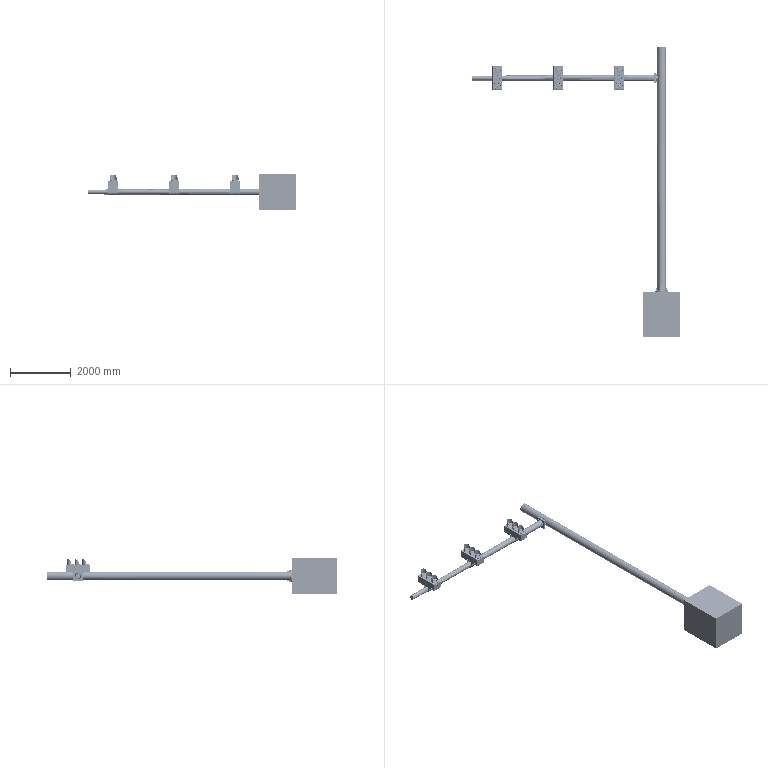Assembly | SolidWorks | mm | 155 component files | 155 solids | 5469 faces | box 6816.5 x 9530 x 1200 mm | volume 2287948976 mm3 | cylinder 2731 | plane 1552 | cone 624 | spline 470 | torus 92 | commonest cylinder face diameters 5 x1476 8 x192 9 x180 10 x168 6 x108 2 x72 15 x72 7 x72
Bill of materials:
Accessory1 | 3 |  | U-shaped thin-wall channel or saddle: a semicircular trough with straight vertical side walls ending in two flat outward flanges, each with two small through-holes.
Base | 1 |  | Plain rectangular block with a row of small cylindrical pins sticking out of one face.
Cantilever | 1 |  | Long, slender round tube with a square end plate at one end. The plate has a central circular opening and four corner holes.
Cap | 1 |  | Short cylindrical cup or cap: a thin-walled ring closed at one end by a flat disc.
Column | 1 |  | Long round tube with a circular bolt-hole flange at one end and a small rectangular tab or bracket plate attached near the other end.
GB_T5786-2000[HexHeadBoltFineThreadFullThreadM16_1.5_70] | 4 |  | Hex-head bolt-like part: a hexagonal head with a long, plain cylindrical shank. The shank's free end is chamfered.
GB_T6170-2015[Type1HexNutM16] | 4 |  | Hex nut-like part: a hexagonal prism with a central through-bore and chamfered corners on both faces.
GB_T6170-2015[Type1HexNutM24] | 8 |  | Hex nut-like part: a hexagonal prism with a central through-bore and double-sided corner chamfers. It looks almost the same as unnamed part.
HexFlangeBoltM10x25 | 12 |  | Hex flange-head bolt or screw: a hexagonal head with an integral round flange washer and a plain cylindrical shank.
HexNutM10 | 12 |  | Hexagonal nut with a plain central through-bore and chamfered corners on both faces.
CoverPlate | 3 |  | Shallow rectangular tray or pan: a flat base with a low wall around all four sides and several through-holes in the base.
GreenLight | 3 |  | Round cap or plug: a slightly domed disc with a thin rim, over a tapered underside that steps down to a smaller cylindrical spigot.
LampHolderMountingPlate | 36 |  | Bent sheet bracket or gusset: a roughly trapezoidal or pentagonal flat plate with one large hole, plus a narrow flange bent up along one curved edge.
Lampshade | 9 |  | Thin curved sheet shroud: a partial cylinder (open arc of about 180-200 degrees) with a curved, sloped top edge and small holes near the bottom edge.
LightBox | 3 |  | Rectangular box-shaped housing. The top face has three large round openings, each surrounded by a pattern of small holes. One end face has a round boss with a hole. The edges are slightly rounded, and there is a recessed lip or panel at the base.
LightMountingPlate | 9 |  | Flat annular ring (washer/flange-like) with four evenly spaced axial through holes, a small radial pin protruding from the outer rim, and a small radial hole in the outer cylindrical face.
OuterFrame | 3 |  | Thin, flat rectangular open frame made of four narrow rails of the same width around a large rectangular opening; the outline is roughly 2.7 times as long as it is wide.
RedLight | 3 |  | Round cap or knob-like solid: a slightly domed top face, a thin cylindrical rim, an underside that curves and tapers inward, and a smaller cylindrical boss at the bottom.
Screw1 | 36 |  | Stepped, rotationally symmetric part: a hollow cylindrical tip with an open bore at the top, a middle step, a larger cylindrical collar, a short plain neck, and a threaded shank modelled with visible thread grooves.
YellowLight | 3 |  | Round cap or knob-like solid: a slightly domed top face, a thin cylindrical rim, an underside that curves and tapers inward, and a cylindrical boss at the bottom.
Mates:
1. concentric | Column-1 face at (-142.894, -198, 82.5) dir (0, 1, 0) r 12 | Base-1 face at (-142.894, 50, 82.5) dir (0, -1, 0) r 12
2. concentric | Column-1 face at (-42.705, -198, 159.378) dir (0, 1, 0) r 12 | Base-1 face at (-42.705, 50, 159.378) dir (0, -1, 0) r 12
3. coincident | Column-1 face at (0, 0, 0) dir (0, -1, 0) | Base-1 face at (0, 0, 0) dir (0, 1, 0)
4. coincident | Column-1 face at (0, 20, 0) dir (0, 1, 0) | GB_T6170-2015[Type1HexNutM24]-1 face at (-142.894, 20, 61.715) dir (0, -1, 0)
5. concentric | Cantilever-1 face at (-6216.5, 7000, 0) dir (-1, 0, 0) r 4.667 | Column-1 face at (206.501, 7000, 0) dir (-1, 0, 0) r 80
6. concentric | Column-1 face at (-186.5, 7106.066, 106.066) dir (-1, 0, 0) r 8 | Cantilever-1 face at (-216.5, 7106.066, 106.066) dir (-1, 0, 0) r 8
7. coincident | Column-1 face at (-216.5, 0, 0) dir (-1, 0, 0) | Cantilever-1 face at (-216.5, 7000, 0) dir (1, 0, 0)
8. concentric | Column-1 face at (-186.5, 7106.066, 106.066) dir (-1, 0, 0) r 8 | GB_T5786-2000[HexHeadBoltFineThreadFullThreadM16_1.5_70]-1 face at (-176.5, 7106.066, 106.066) dir (1, 0, 0) r 8
9. coincident | Column-1 face at (-186.5, 0, 0) dir (1, 0, 0) | GB_T5786-2000[HexHeadBoltFineThreadFullThreadM16_1.5_70]-1 face at (-186.5, 7128.247, 115.23) dir (-1, 0, 0)
10. coincident | Cantilever-1 face at (-236.5, 2747.057, -6675.305) dir (-1, 0, 0) | GB_T6170-2015[Type1HexNutM16]-1 face at (-236.5, 7119.922, 106.066) dir (1, 0, 0)
11. concentric | Column-1 face at (0, 8020, 0) dir (0, -1, 0) r 136.5 | Cap-1 face at (0, 7920, 0) dir (0, 1, 0) r 146.5
12. coincident | Column-1 face at (0, 8020, 0) dir (0, 1, 0) | Cap-1 face at (0, 8020, 0) dir (0, -1, 0)
13. parallel | Cap-1 face at (0, 8030, 0) dir (0, 1, 0) | Light-1/LightBox-1 face at (-5543.393, 7384.024, 358.679) dir (0, 1, 0)
14. parallel | Base-1 face at (-600, -1500, -600) dir (0, 0, -1) | Light-1/CoverPlate-1 face at (-5543.955, 7380.024, 119.592) dir (0, 0, -1)
15. concentric | Light-1/CoverPlate-1 face at (-5301.127, 7146.665, 489.592) dir (0, 0, -1) r 5 | Accessory1-1 face at (-5301.127, 7146.665, 479.592) dir (0, 0, -1) r 5
16. coincident | Light-1/CoverPlate-1 face at (-5543.955, 7380.024, 119.592) dir (0, 0, -1) | Accessory1-1 face at (-5123.37, 7112.081, 119.592) dir (0, 0, 1)
17. coincident | Accessory1-1 face at (-5162.522, 7112.081, 109.592) dir (0, 0, -1) | HexFlangeBoltM10x25-1 plane at (-5489.995, 7146.665, 109.592) dir (0, 0, 1)
18. concentric | Accessory1-1 face at (-5489.995, 7146.665, 479.592) dir (0, 0, -1) r 5 | HexFlangeBoltM10x25-1 axis at (-5489.995, 7146.665, 109.592) dir (0, 0, 1)
19. coincident | Accessory1-1 face at (-5162.522, 7112.081, 109.592) dir (0, 0, -1) | HexFlangeBoltM10x25-2 plane at (-5301.127, 7146.665, 109.592) dir (0, 0, 1)
20. concentric | Accessory1-1 face at (-5301.127, 7146.665, 479.592) dir (0, 0, -1) r 5 | HexFlangeBoltM10x25-2 axis at (-5301.127, 7146.665, 109.592) dir (0, 0, 1)
21. coincident | Accessory1-1 face at (-5162.522, 7112.081, 109.592) dir (0, 0, -1) | HexFlangeBoltM10x25-3 plane at (-5301.127, 6853.335, 109.592) dir (0, 0, 1)
22. concentric | Accessory1-1 face at (-5301.127, 6853.335, 479.592) dir (0, 0, -1) r 5 | HexFlangeBoltM10x25-3 axis at (-5301.127, 6853.335, 109.592) dir (0, 0, 1)
23. coincident | Accessory1-1 face at (-5162.522, 7112.081, 109.592) dir (0, 0, -1) | HexFlangeBoltM10x25-4 plane at (-5489.995, 6853.335, 109.592) dir (0, 0, 1)
24. concentric | Accessory1-1 face at (-5489.995, 6853.335, 479.592) dir (0, 0, -1) r 5 | HexFlangeBoltM10x25-4 axis at (-5489.995, 6853.335, 109.592) dir (0, 0, 1)
25. coincident | Accessory1-2 face at (-3162.522, 7112.081, 109.592) dir (0, 0, -1) | HexFlangeBoltM10x25-5 plane at (-3489.995, 7146.665, 109.592) dir (0, 0, 1)
26. concentric | Accessory1-2 face at (-3489.995, 7146.665, 479.592) dir (0, 0, -1) r 5 | HexFlangeBoltM10x25-5 axis at (-3489.995, 7146.665, 109.592) dir (0, 0, 1)
27. coincident | Accessory1-2 face at (-3162.522, 7112.081, 109.592) dir (0, 0, -1) | HexFlangeBoltM10x25-6 plane at (-3301.127, 7146.665, 109.592) dir (0, 0, 1)
28. concentric | Accessory1-2 face at (-3301.127, 7146.665, 479.592) dir (0, 0, -1) r 5 | HexFlangeBoltM10x25-6 axis at (-3301.127, 7146.665, 109.592) dir (0, 0, 1)
29. coincident | Accessory1-2 face at (-3162.522, 7112.081, 109.592) dir (0, 0, -1) | HexFlangeBoltM10x25-7 plane at (-3301.127, 6853.335, 109.592) dir (0, 0, 1)
30. concentric | Accessory1-2 face at (-3301.127, 6853.335, 479.592) dir (0, 0, -1) r 5 | HexFlangeBoltM10x25-7 axis at (-3301.127, 6853.335, 109.592) dir (0, 0, 1)
31. coincident | Accessory1-2 face at (-3162.522, 7112.081, 109.592) dir (0, 0, -1) | HexFlangeBoltM10x25-8 plane at (-3489.995, 6853.335, 109.592) dir (0, 0, 1)
32. concentric | Accessory1-2 face at (-3489.995, 6853.335, 479.592) dir (0, 0, -1) r 5 | HexFlangeBoltM10x25-8 axis at (-3489.995, 6853.335, 109.592) dir (0, 0, 1)
33. coincident | Accessory1-3 face at (-1162.522, 7112.081, 109.592) dir (0, 0, -1) | HexFlangeBoltM10x25-9 plane at (-1489.995, 7146.665, 109.592) dir (0, 0, 1)
34. concentric | Accessory1-3 face at (-1489.995, 7146.665, 479.592) dir (0, 0, -1) r 5 | HexFlangeBoltM10x25-9 axis at (-1489.995, 7146.665, 109.592) dir (0, 0, 1)
35. coincident | Accessory1-3 face at (-1162.522, 7112.081, 109.592) dir (0, 0, -1) | HexFlangeBoltM10x25-10 plane at (-1301.127, 7146.665, 109.592) dir (0, 0, 1)
36. concentric | Accessory1-3 face at (-1301.127, 7146.665, 479.592) dir (0, 0, -1) r 5 | HexFlangeBoltM10x25-10 axis at (-1301.127, 7146.665, 109.592) dir (0, 0, 1)
37. coincident | Accessory1-3 face at (-1162.522, 7112.081, 109.592) dir (0, 0, -1) | HexFlangeBoltM10x25-11 plane at (-1301.127, 6853.335, 109.592) dir (0, 0, 1)
38. concentric | Accessory1-3 face at (-1301.127, 6853.335, 479.592) dir (0, 0, -1) r 5 | HexFlangeBoltM10x25-11 axis at (-1301.127, 6853.335, 109.592) dir (0, 0, 1)
39. coincident | Accessory1-3 face at (-1162.522, 7112.081, 109.592) dir (0, 0, -1) | HexFlangeBoltM10x25-12 plane at (-1489.995, 6853.335, 109.592) dir (0, 0, 1)
40. concentric | Accessory1-3 face at (-1489.995, 6853.335, 479.592) dir (0, 0, -1) r 5 | HexFlangeBoltM10x25-12 axis at (-1489.995, 6853.335, 109.592) dir (0, 0, 1)
41. coincident | Light-1/CoverPlate-1 face at (-5543.955, 7380.024, 122.592) dir (0, 0, 1) | HexNutM10-10 plane at (-5301.127, 7146.665, 122.592) dir (0, 0, -1)
42. concentric | HexFlangeBoltM10x25-2 face at (-5301.127, 7146.665, 134.592) dir (0, 0, -1) r 5 | HexNutM10-10 axis at (-5301.127, 7146.665, 122.592) dir (0, 0, 1)
43. coincident | Light-1/CoverPlate-1 face at (-5543.955, 7380.024, 122.592) dir (0, 0, 1) | HexNutM10-11 plane at (-5489.995, 7146.665, 122.592) dir (0, 0, -1)
44. concentric | HexFlangeBoltM10x25-1 face at (-5489.995, 7146.665, 134.592) dir (0, 0, -1) r 5 | HexNutM10-11 axis at (-5489.995, 7146.665, 122.592) dir (0, 0, 1)
45. coincident | Light-1/CoverPlate-1 face at (-5543.955, 7380.024, 122.592) dir (0, 0, 1) | HexNutM10-12 plane at (-5489.995, 6853.335, 122.592) dir (0, 0, -1)
46. concentric | HexFlangeBoltM10x25-4 face at (-5489.995, 6853.335, 134.592) dir (0, 0, -1) r 5 | HexNutM10-12 axis at (-5489.995, 6853.335, 122.592) dir (0, 0, 1)
47. coincident | Light-1/CoverPlate-1 face at (-5543.955, 7380.024, 122.592) dir (0, 0, 1) | HexNutM10-13 plane at (-5301.127, 6853.335, 122.592) dir (0, 0, -1)
48. concentric | HexFlangeBoltM10x25-3 face at (-5301.127, 6853.335, 134.592) dir (0, 0, -1) r 5 | HexNutM10-13 axis at (-5301.127, 6853.335, 122.592) dir (0, 0, 1)
49. coincident | Light-2/CoverPlate-1 face at (-3543.955, 7380.024, 122.592) dir (0, 0, 1) | HexNutM10-14 plane at (-3489.995, 7146.665, 122.592) dir (0, 0, -1)
50. concentric | HexFlangeBoltM10x25-5 face at (-3489.995, 7146.665, 134.592) dir (0, 0, -1) r 5 | HexNutM10-14 axis at (-3489.995, 7146.665, 122.592) dir (0, 0, 1)
51. coincident | Light-2/CoverPlate-1 face at (-3543.955, 7380.024, 122.592) dir (0, 0, 1) | HexNutM10-15 plane at (-3301.127, 7146.665, 122.592) dir (0, 0, -1)
52. concentric | HexFlangeBoltM10x25-6 face at (-3301.127, 7146.665, 134.592) dir (0, 0, -1) r 5 | HexNutM10-15 axis at (-3301.127, 7146.665, 122.592) dir (0, 0, 1)
53. coincident | Light-2/CoverPlate-1 face at (-3543.955, 7380.024, 122.592) dir (0, 0, 1) | HexNutM10-16 plane at (-3301.127, 6853.335, 122.592) dir (0, 0, -1)
54. concentric | HexFlangeBoltM10x25-7 face at (-3301.127, 6853.335, 134.592) dir (0, 0, -1) r 5 | HexNutM10-16 axis at (-3301.127, 6853.335, 122.592) dir (0, 0, 1)
55. coincident | Light-2/CoverPlate-1 face at (-3543.955, 7380.024, 122.592) dir (0, 0, 1) | HexNutM10-17 plane at (-3489.995, 6853.335, 122.592) dir (0, 0, -1)
56. concentric | HexFlangeBoltM10x25-8 face at (-3489.995, 6853.335, 134.592) dir (0, 0, -1) r 5 | HexNutM10-17 axis at (-3489.995, 6853.335, 122.592) dir (0, 0, 1)
57. coincident | Light-3/CoverPlate-1 face at (-1543.955, 7380.024, 122.592) dir (0, 0, 1) | HexNutM10-18 plane at (-1489.995, 7146.665, 122.592) dir (0, 0, -1)
58. concentric | HexFlangeBoltM10x25-9 face at (-1489.995, 7146.665, 134.592) dir (0, 0, -1) r 5 | HexNutM10-18 axis at (-1489.995, 7146.665, 122.592) dir (0, 0, 1)
59. coincident | Light-3/CoverPlate-1 face at (-1543.955, 7380.024, 122.592) dir (0, 0, 1) | HexNutM10-19 plane at (-1301.127, 7146.665, 122.592) dir (0, 0, -1)
60. concentric | HexFlangeBoltM10x25-10 face at (-1301.127, 7146.665, 134.592) dir (0, 0, -1) r 5 | HexNutM10-19 axis at (-1301.127, 7146.665, 122.592) dir (0, 0, 1)
61. coincident | Light-3/CoverPlate-1 face at (-1543.955, 7380.024, 122.592) dir (0, 0, 1) | HexNutM10-20 plane at (-1301.127, 6853.335, 122.592) dir (0, 0, -1)
62. concentric | HexFlangeBoltM10x25-11 face at (-1301.127, 6853.335, 134.592) dir (0, 0, -1) r 5 | HexNutM10-20 axis at (-1301.127, 6853.335, 122.592) dir (0, 0, 1)
63. coincident | Light-3/CoverPlate-1 face at (-1543.955, 7380.024, 122.592) dir (0, 0, 1) | HexNutM10-21 plane at (-1489.995, 6853.335, 122.592) dir (0, 0, -1)
64. concentric | HexFlangeBoltM10x25-12 face at (-1489.995, 6853.335, 134.592) dir (0, 0, -1) r 5 | HexNutM10-21 axis at (-1489.995, 6853.335, 122.592) dir (0, 0, 1)
65. concentric | Base-1 face at (-142.894, 50, 82.5) dir (0, -1, 0) r 12 | GB_T6170-2015[Type1HexNutM24]-1 face at (-142.894, 20, 82.5) dir (0, 1, 0) r 12
66. concentric | GB_T5786-2000[HexHeadBoltFineThreadFullThreadM16_1.5_70]-1 face at (-176.5, 7106.066, 106.066) dir (1, 0, 0) r 8 | GB_T6170-2015[Type1HexNutM16]-1 face at (-236.5, 7106.066, 106.066) dir (-1, 0, 0) r 8